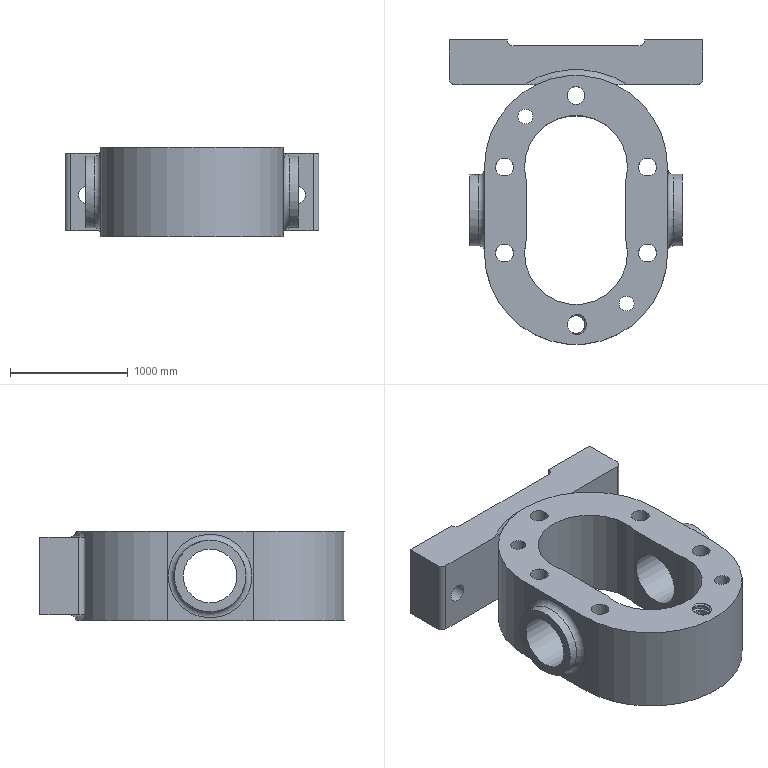Component | NX | 6 | 1 solid | 47 faces | volume 1660576720 mm3 | cylinder 24 | plane 17 | torus 4 | spline 2 | commonest cylinder face diameters 152.4 x8 101.6 x4 1555.496 x3 876.3 x2 609.6 x2 457.2 x2 127 x2 177.8 x1